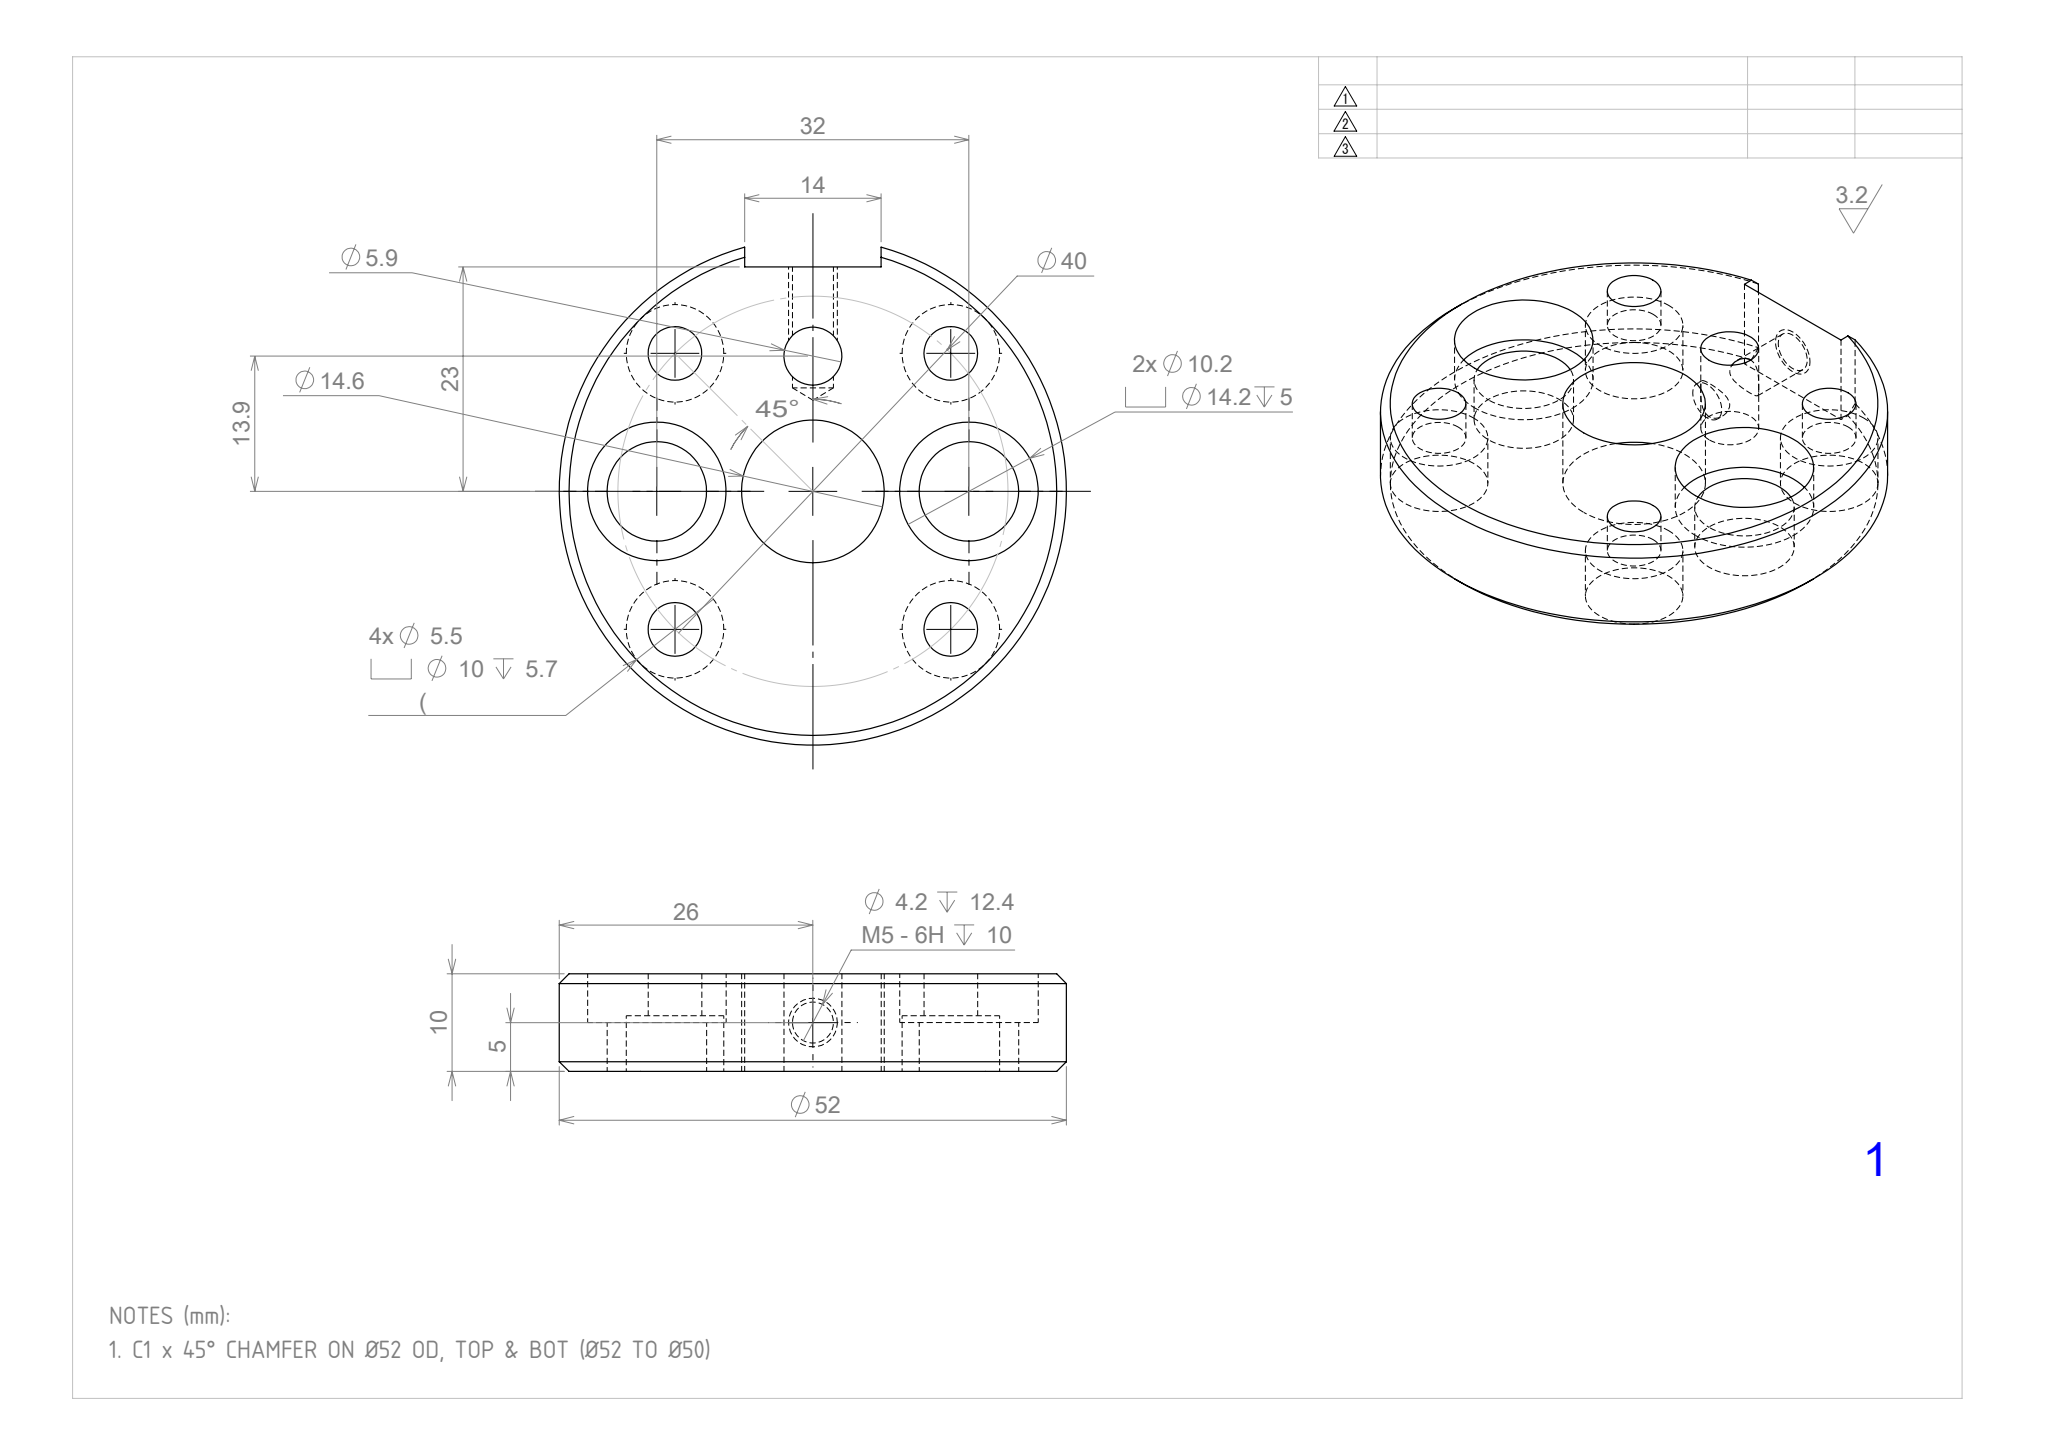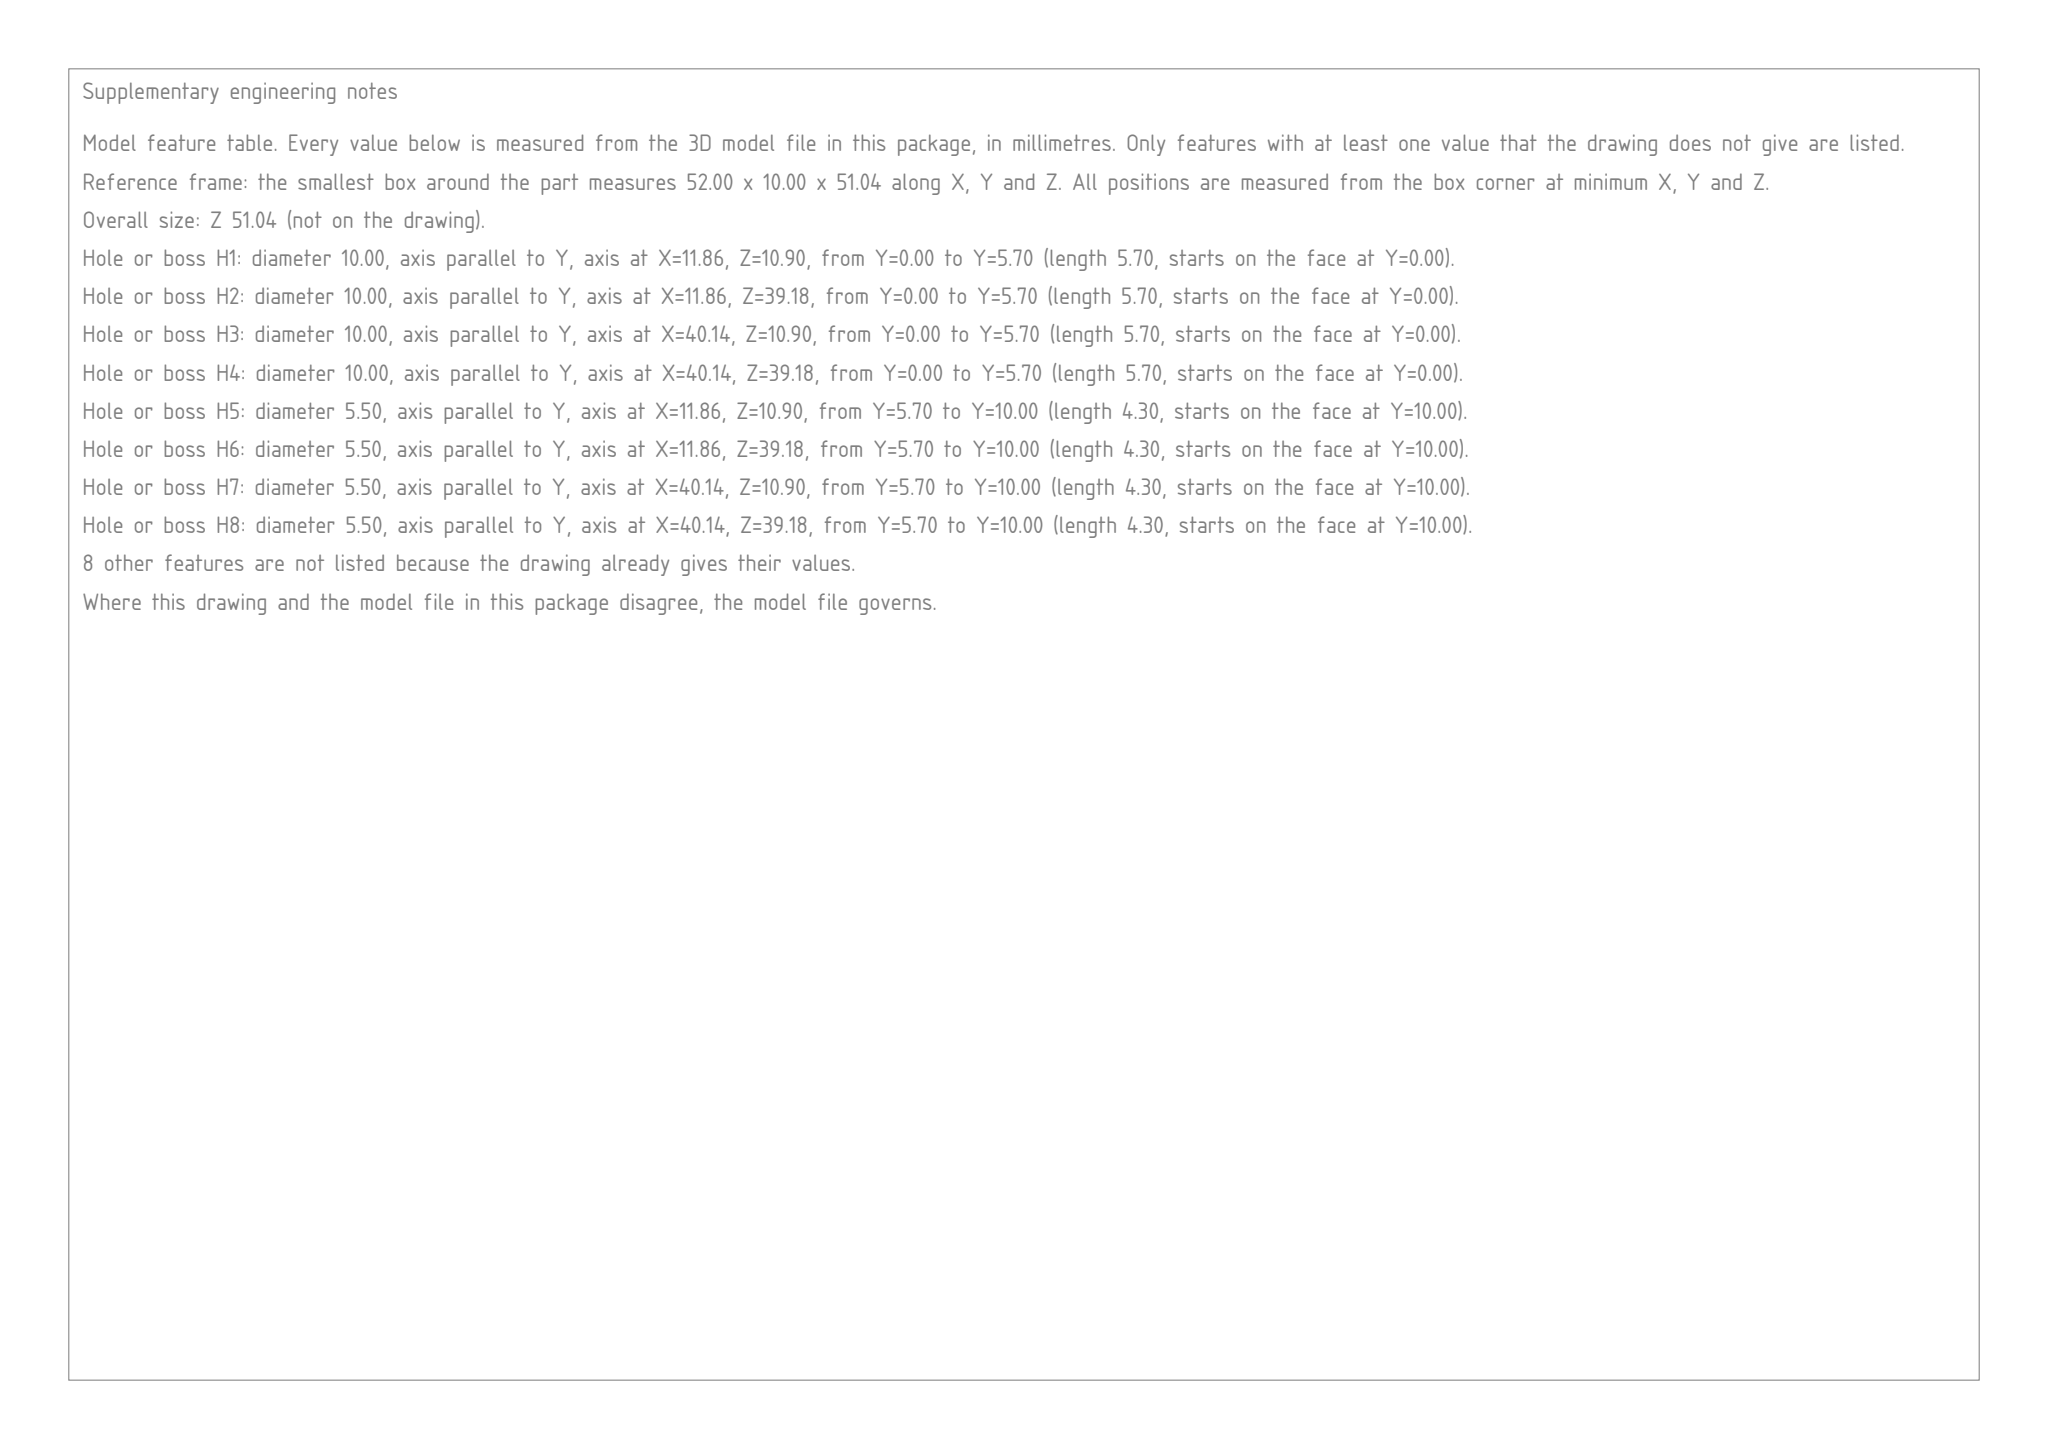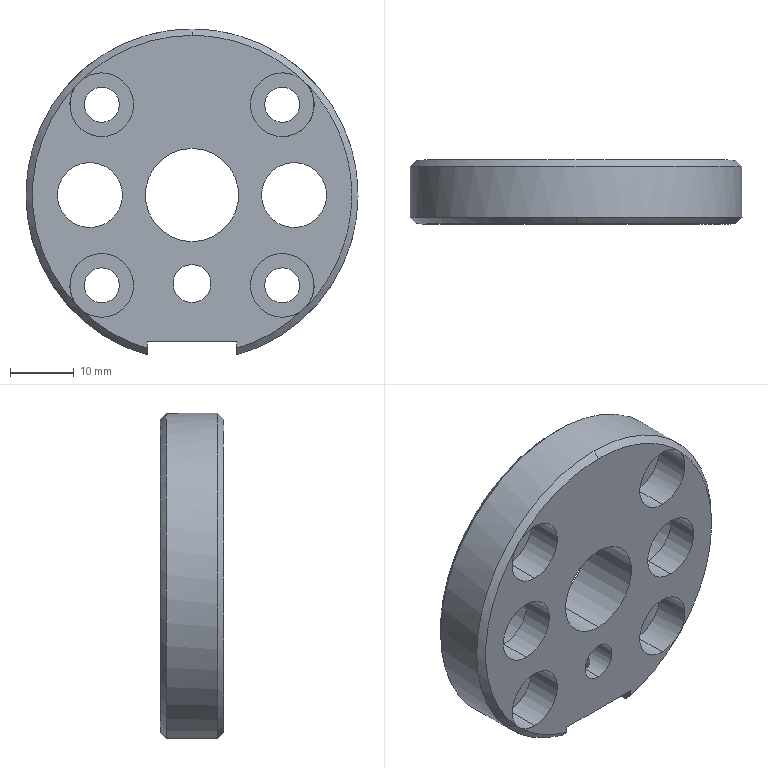Part | SolidWorks | mm | 1 solid | 49 faces | box 52 x 10 x 51.04 mm | volume 14058 mm3 | cylinder 33 | plane 11 | cone 5 | commonest cylinder face diameters 10 x8 5.5 x8 4.2 x4 14.2 x4 10.2 x4 14.62 x2 5.939 x2 52 x1
Drawing notes:
C1 x 45° CHAMFER ON Ø52 OD, TOP & BOT (Ø52 TO Ø50) | from the solid: cones[90,52]x2 and [90,50]x1 on Ø52 OD; 90° incl = 45° x 1 per side